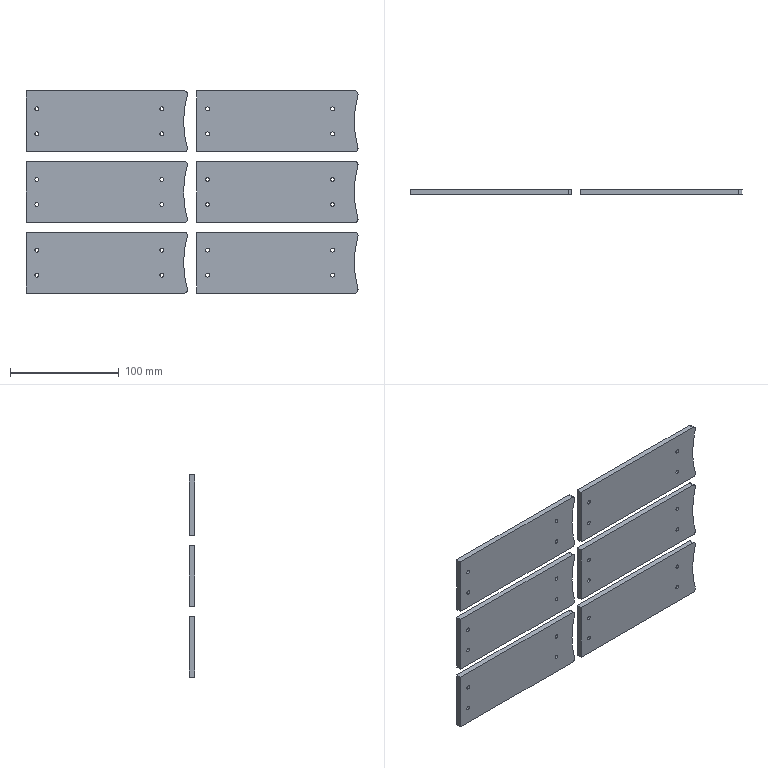CAM job | Mastercam | mm | 4 operations | part box 305.42 x 5 x 186
1. Contour (Ramp) | 3 - 3 平铣刀
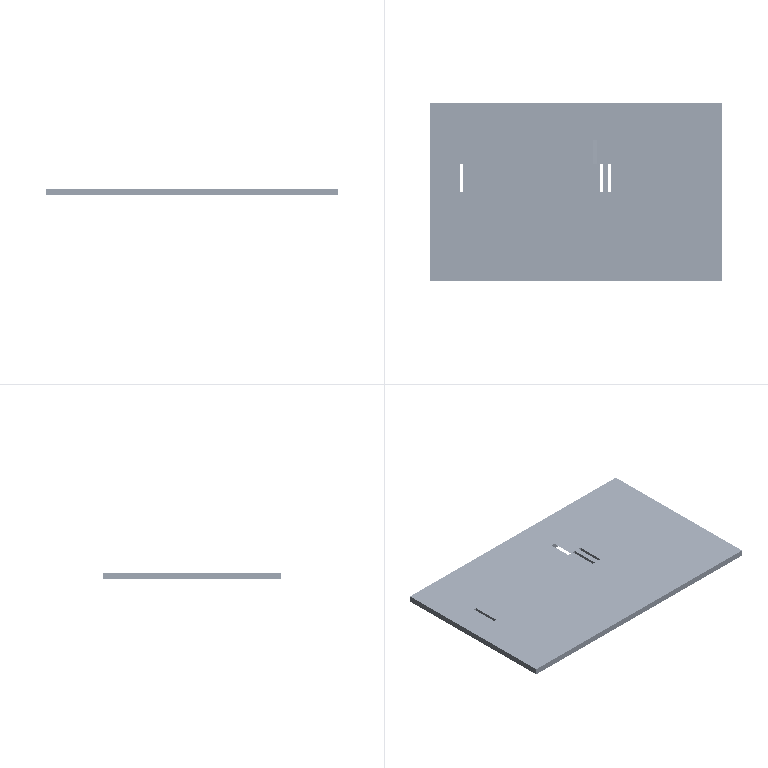2. Contour (2D chamfer) | 7 - 4 倒角刀
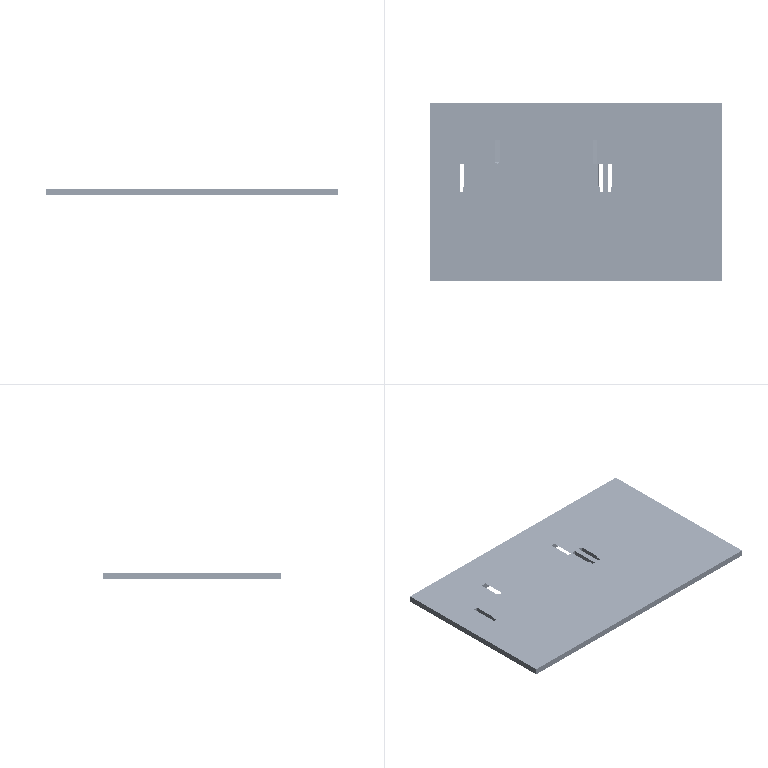3. Drill/Counterbore | 7 - 4 倒角刀
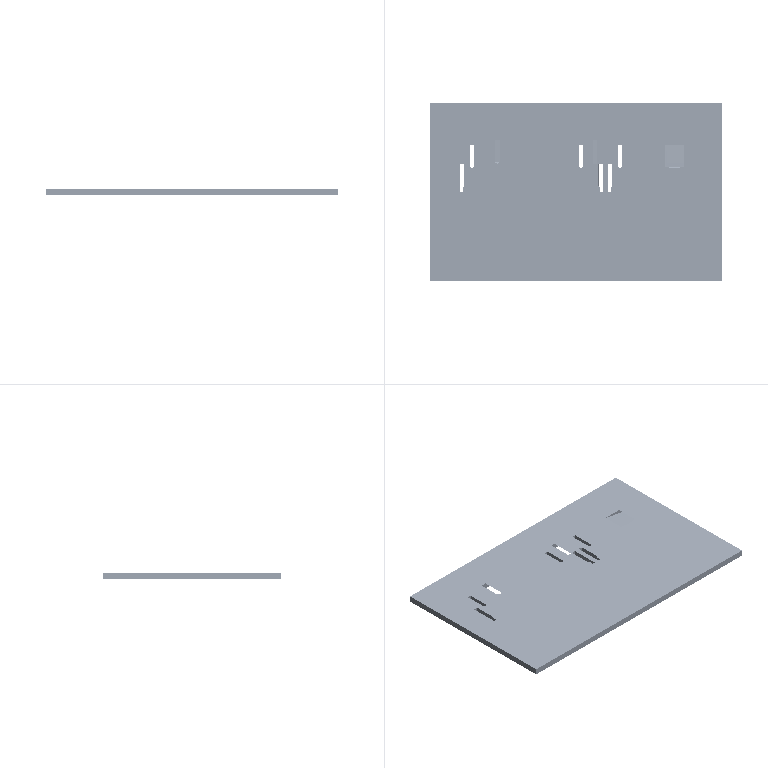4. Contour (Ramp) | 2 - 2 平铣刀